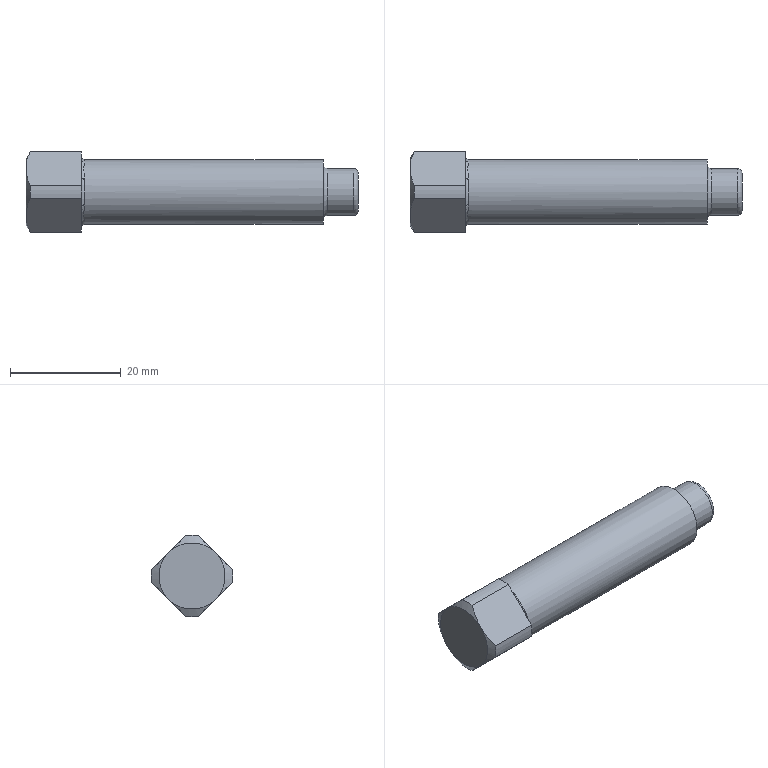Component | NX | GB85-88_M12X50 | 1 solid | 31 faces | volume 6437 mm3 | plane 11 | cylinder 6 | torus 6 | cone 4 | spline 4 | commonest cylinder face diameters 14.7 x4 8.5 x1 11.701 x1